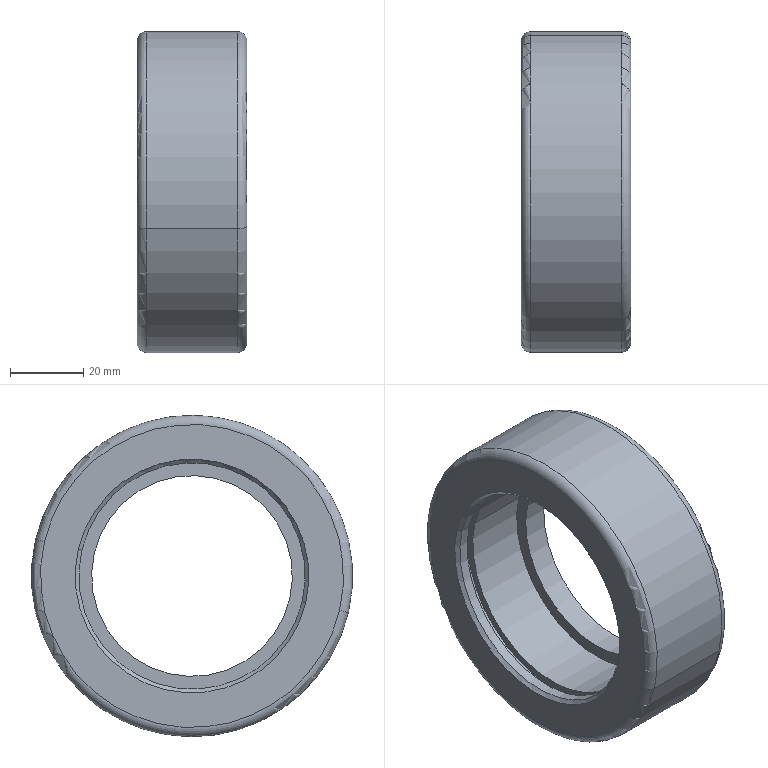Component | SolidWorks | GuideWheelAssembly-1_GuideWheel-2 | 1 solid | 21 faces | box 30 x 88 x 88 mm | volume 94633 mm3 | cylinder 10 | plane 5 | torus 4 | cone 2 | commonest cylinder face diameters 62 x4 66.2 x2 55 x2 88 x2 | material Nylon 101
build123d program:
from build123d import *

# Parameters (mm, degrees)
SKETCH1_R           = 44
BOSS_EXTRUDE1_DEPTH = 30
SKETCH4_R           = 31
CUT_EXTRUDE2_DEPTH  = 67.34
SKETCH5_R           = 27.5
CUT_EXTRUDE3_DEPTH  = 70.08
SKETCH6_R           = 33.1
CUT_EXTRUDE4_DEPTH  = 2.2
CHAMFER1_SIZE       = 1
FILLET1_R           = 2.5


with BuildPart() as part:
    # Sketch1 → Boss-Extrude1 (new body)
    with BuildSketch(Plane.XY):
        Circle(SKETCH1_R)
    extrude(amount=BOSS_EXTRUDE1_DEPTH)

    # Sketch4 → Cut-Extrude2 (cut, through all)
    with BuildSketch(Plane.XY.offset(7)):
        Circle(SKETCH4_R)
    extrude(amount=CUT_EXTRUDE2_DEPTH, mode=Mode.SUBTRACT)

    # Sketch5 → Cut-Extrude3 (cut, through all)
    with BuildSketch(Plane(origin=(0, 0, 0), x_dir=(-1, 0, 0), z_dir=(0, 0, -1))):
        Circle(SKETCH5_R)
    extrude(amount=-CUT_EXTRUDE3_DEPTH, mode=Mode.SUBTRACT)

    # Sketch6 → Cut-Extrude4 (cut)
    with BuildSketch(Plane.XY.offset(24)):
        Circle(SKETCH6_R)
    extrude(amount=CUT_EXTRUDE4_DEPTH, mode=Mode.SUBTRACT)

    # Chamfer1
    chamfer1_edges = [part.edges().sort_by_distance(p)[0] for p in [
        (-31, 0, 30),
    ]]
    chamfer(chamfer1_edges, length=CHAMFER1_SIZE)

    # Fillet1
    fillet1_edges = [part.edges().sort_by_distance(p)[0] for p in [
        (-44, 0, 0),
        (-44, 0, 30),
    ]]
    fillet(fillet1_edges, radius=FILLET1_R)


solid = part.part

# Placed as in the assembly
solid = solid.moved(Location((-540, 0, 25), (0, -90, 0)))
STEP:
#1=COLOUR_RGB('',0.7922,0.8196,0.9333);
#2=FILL_AREA_STYLE_COLOUR('',#1);
#3=FILL_AREA_STYLE('',(#2));
#4=SURFACE_STYLE_FILL_AREA(#3);
#5=SURFACE_SIDE_STYLE('',(#4));
#6=SURFACE_STYLE_USAGE(.BOTH.,#5);
#7=PRESENTATION_STYLE_ASSIGNMENT((#6));
#8=CARTESIAN_POINT('',(-21.26,-1.591,0.6126));
#9=VERTEX_POINT('',#8);
#10=CARTESIAN_POINT('',(-21.26,1.591,1.356));
#11=VERTEX_POINT('',#10);
#12=CARTESIAN_POINT('',(-21.26,-0.,0.9843));
#13=DIRECTION('',(1.,0.,0.));
#14=DIRECTION('',(0.,0.9738,0.2275));
#15=AXIS2_PLACEMENT_3D('',#12,#13,#14);
#16=CIRCLE('',#15,1.634);
#17=EDGE_CURVE('',#9,#11,#16,.T.);
#18=ORIENTED_EDGE('',*,*,#17,.F.);
#19=CARTESIAN_POINT('',(-21.358,-1.687,0.5902));
#20=VERTEX_POINT('',#19);
#21=CARTESIAN_POINT('',(-21.358,-1.591,0.6126));
#22=DIRECTION('',(0.,0.2275,-0.9738));
#23=DIRECTION('',(0.,0.9738,0.2275));
#24=AXIS2_PLACEMENT_3D('',#21,#22,#23);
#25=CIRCLE('',#24,0.09843);
#26=EDGE_CURVE('',#9,#20,#25,.T.);
#27=ORIENTED_EDGE('',*,*,#26,.T.);
#28=CARTESIAN_POINT('',(-21.358,1.687,1.378));
#29=VERTEX_POINT('',#28);
#30=CARTESIAN_POINT('',(-21.358,-0.,0.9843));
#31=DIRECTION('',(-1.,0.,0.));
#32=DIRECTION('',(0.,0.9738,0.2275));
#33=AXIS2_PLACEMENT_3D('',#30,#31,#32);
#34=CIRCLE('',#33,1.732);
#35=EDGE_CURVE('',#29,#20,#34,.T.);
#36=ORIENTED_EDGE('',*,*,#35,.F.);
#37=CARTESIAN_POINT('',(-21.358,1.591,1.356));
#38=DIRECTION('',(0.,-0.2275,0.9738));
#39=DIRECTION('',(0.,-0.9738,-0.2275));
#40=AXIS2_PLACEMENT_3D('',#37,#38,#39);
#41=CIRCLE('',#40,0.09843);
#42=EDGE_CURVE('',#11,#29,#41,.T.);
#43=ORIENTED_EDGE('',*,*,#42,.F.);
#44=EDGE_LOOP('',(#18,#27,#36,#43));
#45=FACE_OUTER_BOUND('',#44,.T.);
#46=CARTESIAN_POINT('',(-21.358,-0.,0.9843));
#47=DIRECTION('',(-1.,0.,0.));
#48=DIRECTION('',(0.,0.9738,0.2275));
#49=AXIS2_PLACEMENT_3D('',#46,#47,#48);
#50=TOROIDAL_SURFACE('',#49,1.634,0.09843);
#51=ADVANCED_FACE('',(#45),#50,.T.);
#52=CARTESIAN_POINT('',(-22.343,-1.687,0.5902));
#53=VERTEX_POINT('',#52);
#54=CARTESIAN_POINT('',(-22.343,1.687,1.378));
#55=VERTEX_POINT('',#54);
#56=CARTESIAN_POINT('',(-22.343,-0.,0.9843));
#57=DIRECTION('',(1.,0.,0.));
#58=DIRECTION('',(0.,0.9738,0.2275));
#59=AXIS2_PLACEMENT_3D('',#56,#57,#58);
#60=CIRCLE('',#59,1.732);
#61=EDGE_CURVE('',#53,#55,#60,.T.);
#62=ORIENTED_EDGE('',*,*,#61,.F.);
#63=CARTESIAN_POINT('',(-22.441,-1.591,0.6126));
#64=VERTEX_POINT('',#63);
#65=CARTESIAN_POINT('',(-22.343,-1.591,0.6126));
#66=DIRECTION('',(0.,0.2275,-0.9738));
#67=DIRECTION('',(0.,0.9738,0.2275));
#68=AXIS2_PLACEMENT_3D('',#65,#66,#67);
#69=CIRCLE('',#68,0.09843);
#70=EDGE_CURVE('',#53,#64,#69,.T.);
#71=ORIENTED_EDGE('',*,*,#70,.T.);
#72=CARTESIAN_POINT('',(-22.441,1.591,1.356));
#73=VERTEX_POINT('',#72);
#74=CARTESIAN_POINT('',(-22.441,-0.,0.9843));
#75=DIRECTION('',(-1.,0.,0.));
#76=DIRECTION('',(0.,0.9738,0.2275));
#77=AXIS2_PLACEMENT_3D('',#74,#75,#76);
#78=CIRCLE('',#77,1.634);
#79=EDGE_CURVE('',#73,#64,#78,.T.);
#80=ORIENTED_EDGE('',*,*,#79,.F.);
#81=CARTESIAN_POINT('',(-22.343,1.591,1.356));
#82=DIRECTION('',(0.,-0.2275,0.9738));
#83=DIRECTION('',(0.,-0.9738,-0.2275));
#84=AXIS2_PLACEMENT_3D('',#81,#82,#83);
#85=CIRCLE('',#84,0.09843);
#86=EDGE_CURVE('',#55,#73,#85,.T.);
#87=ORIENTED_EDGE('',*,*,#86,.F.);
#88=EDGE_LOOP('',(#62,#71,#80,#87));
#89=FACE_OUTER_BOUND('',#88,.T.);
#90=CARTESIAN_POINT('',(-22.343,-0.,0.9843));
#91=DIRECTION('',(-1.,0.,0.));
#92=DIRECTION('',(0.,0.9738,0.2275));
#93=AXIS2_PLACEMENT_3D('',#90,#91,#92);
#94=TOROIDAL_SURFACE('',#93,1.634,0.09843);
#95=ADVANCED_FACE('',(#89),#94,.T.);
#96=CARTESIAN_POINT('',(-22.402,-1.188,0.7066));
#97=VERTEX_POINT('',#96);
#98=CARTESIAN_POINT('',(-22.402,1.188,1.262));
#99=VERTEX_POINT('',#98);
#100=CARTESIAN_POINT('',(-22.402,-0.,0.9843));
#101=DIRECTION('',(-1.,0.,0.));
#102=DIRECTION('',(0.,0.9738,0.2275));
#103=AXIS2_PLACEMENT_3D('',#100,#101,#102);
#104=CIRCLE('',#103,1.22);
#105=EDGE_CURVE('',#97,#99,#104,.T.);
#106=ORIENTED_EDGE('',*,*,#105,.F.);
#107=CARTESIAN_POINT('',(-22.441,-1.227,0.6977));
#108=VERTEX_POINT('',#107);
#109=CARTESIAN_POINT('',(-22.402,-1.188,0.7066));
#110=DIRECTION('',(-0.7071,-0.6886,-0.1608));
#111=VECTOR('',#110,39.37);
#112=LINE('',#109,#111);
#113=EDGE_CURVE('',#97,#108,#112,.T.);
#114=ORIENTED_EDGE('',*,*,#113,.T.);
#115=CARTESIAN_POINT('',(-22.441,1.227,1.271));
#116=VERTEX_POINT('',#115);
#117=CARTESIAN_POINT('',(-22.441,-0.,0.9843));
#118=DIRECTION('',(1.,0.,0.));
#119=DIRECTION('',(0.,0.9738,0.2275));
#120=AXIS2_PLACEMENT_3D('',#117,#118,#119);
#121=CIRCLE('',#120,1.26);
#122=EDGE_CURVE('',#116,#108,#121,.T.);
#123=ORIENTED_EDGE('',*,*,#122,.F.);
#124=CARTESIAN_POINT('',(-22.402,1.188,1.262));
#125=DIRECTION('',(-0.7071,0.6886,0.1608));
#126=VECTOR('',#125,39.37);
#127=LINE('',#124,#126);
#128=EDGE_CURVE('',#99,#116,#127,.T.);
#129=ORIENTED_EDGE('',*,*,#128,.F.);
#130=EDGE_LOOP('',(#106,#114,#123,#129));
#131=FACE_OUTER_BOUND('',#130,.T.);
#132=CARTESIAN_POINT('',(-22.402,-0.,0.9843));
#133=DIRECTION('',(-1.,0.,0.));
#134=DIRECTION('',(0.,0.9738,0.2275));
#135=AXIS2_PLACEMENT_3D('',#132,#133,#134);
#136=CONICAL_SURFACE('',#135,1.22,0.7854);
#137=ADVANCED_FACE('',(#131),#136,.F.);
#138=CARTESIAN_POINT('',(-22.291,-1.269,0.6878));
#139=VERTEX_POINT('',#138);
#140=CARTESIAN_POINT('',(-22.291,1.269,1.281));
#141=VERTEX_POINT('',#140);
#142=CARTESIAN_POINT('',(-22.291,-0.,0.9843));
#143=DIRECTION('',(-1.,0.,0.));
#144=DIRECTION('',(0.,0.9738,0.2275));
#145=AXIS2_PLACEMENT_3D('',#142,#143,#144);
#146=CIRCLE('',#145,1.303);
#147=EDGE_CURVE('',#139,#141,#146,.T.);
#148=ORIENTED_EDGE('',*,*,#147,.T.);
#149=CARTESIAN_POINT('',(-22.205,1.269,1.281));
#150=VERTEX_POINT('',#149);
#151=CARTESIAN_POINT('',(-22.291,1.269,1.281));
#152=DIRECTION('',(1.,0.,0.));
#153=VECTOR('',#152,39.37);
#154=LINE('',#151,#153);
#155=EDGE_CURVE('',#141,#150,#154,.T.);
#156=ORIENTED_EDGE('',*,*,#155,.T.);
#157=CARTESIAN_POINT('',(-22.205,-1.269,0.6878));
#158=VERTEX_POINT('',#157);
#159=CARTESIAN_POINT('',(-22.205,-0.,0.9843));
#160=DIRECTION('',(-1.,0.,0.));
#161=DIRECTION('',(0.,0.9738,0.2275));
#162=AXIS2_PLACEMENT_3D('',#159,#160,#161);
#163=CIRCLE('',#162,1.303);
#164=EDGE_CURVE('',#158,#150,#163,.T.);
#165=ORIENTED_EDGE('',*,*,#164,.F.);
#166=CARTESIAN_POINT('',(-22.291,-1.269,0.6878));
#167=DIRECTION('',(1.,0.,0.));
#168=VECTOR('',#167,39.37);
#169=LINE('',#166,#168);
#170=EDGE_CURVE('',#139,#158,#169,.T.);
#171=ORIENTED_EDGE('',*,*,#170,.F.);
#172=EDGE_LOOP('',(#148,#156,#165,#171));
#173=FACE_OUTER_BOUND('',#172,.T.);
#174=CARTESIAN_POINT('',(-22.291,-0.,0.9843));
#175=DIRECTION('',(1.,0.,0.));
#176=DIRECTION('',(0.,-0.9738,-0.2275));
#177=AXIS2_PLACEMENT_3D('',#174,#175,#176);
#178=CYLINDRICAL_SURFACE('',#177,1.303);
#179=ADVANCED_FACE('',(#173),#178,.F.);
#180=CARTESIAN_POINT('',(-21.535,-1.054,0.738));
#181=VERTEX_POINT('',#180);
#182=CARTESIAN_POINT('',(-21.535,1.054,1.231));
#183=VERTEX_POINT('',#182);
#184=CARTESIAN_POINT('',(-21.535,-0.,0.9843));
#185=DIRECTION('',(-1.,0.,0.));
#186=DIRECTION('',(0.,0.9738,0.2275));
#187=AXIS2_PLACEMENT_3D('',#184,#185,#186);
#188=CIRCLE('',#187,1.083);
#189=EDGE_CURVE('',#181,#183,#188,.T.);
#190=ORIENTED_EDGE('',*,*,#189,.T.);
#191=CARTESIAN_POINT('',(-21.26,1.054,1.231));
#192=VERTEX_POINT('',#191);
#193=CARTESIAN_POINT('',(-22.441,1.054,1.231));
#194=DIRECTION('',(1.,0.,0.));
#195=VECTOR('',#194,39.37);
#196=LINE('',#193,#195);
#197=EDGE_CURVE('',#183,#192,#196,.T.);
#198=ORIENTED_EDGE('',*,*,#197,.T.);
#199=CARTESIAN_POINT('',(-21.26,-1.054,0.738));
#200=VERTEX_POINT('',#199);
#201=CARTESIAN_POINT('',(-21.26,-0.,0.9843));
#202=DIRECTION('',(1.,0.,0.));
#203=DIRECTION('',(0.,-0.9738,-0.2275));
#204=AXIS2_PLACEMENT_3D('',#201,#202,#203);
#205=CIRCLE('',#204,1.083);
#206=EDGE_CURVE('',#192,#200,#205,.T.);
#207=ORIENTED_EDGE('',*,*,#206,.T.);
#208=CARTESIAN_POINT('',(-22.441,-1.054,0.738));
#209=DIRECTION('',(1.,0.,0.));
#210=VECTOR('',#209,39.37);
#211=LINE('',#208,#210);
#212=EDGE_CURVE('',#181,#200,#211,.T.);
#213=ORIENTED_EDGE('',*,*,#212,.F.);
#214=EDGE_LOOP('',(#190,#198,#207,#213));
#215=FACE_OUTER_BOUND('',#214,.T.);
#216=CARTESIAN_POINT('',(-22.441,-0.,0.9843));
#217=DIRECTION('',(1.,0.,0.));
#218=DIRECTION('',(0.,-0.9738,-0.2275));
#219=AXIS2_PLACEMENT_3D('',#216,#217,#218);
#220=CYLINDRICAL_SURFACE('',#219,1.083);
#221=ADVANCED_FACE('',(#215),#220,.F.);
#222=ORIENTED_EDGE('',*,*,#105,.T.);
#223=CARTESIAN_POINT('',(-22.291,1.188,1.262));
#224=VERTEX_POINT('',#223);
#225=CARTESIAN_POINT('',(-22.441,1.188,1.262));
#226=DIRECTION('',(1.,0.,0.));
#227=VECTOR('',#226,39.37);
#228=LINE('',#225,#227);
#229=EDGE_CURVE('',#99,#224,#228,.T.);
#230=ORIENTED_EDGE('',*,*,#229,.T.);
#231=CARTESIAN_POINT('',(-22.291,-1.188,0.7066));
#232=VERTEX_POINT('',#231);
#233=CARTESIAN_POINT('',(-22.291,-0.,0.9843));
#234=DIRECTION('',(-1.,0.,0.));
#235=DIRECTION('',(0.,0.9738,0.2275));
#236=AXIS2_PLACEMENT_3D('',#233,#234,#235);
#237=CIRCLE('',#236,1.22);
#238=EDGE_CURVE('',#232,#224,#237,.T.);
#239=ORIENTED_EDGE('',*,*,#238,.F.);
#240=CARTESIAN_POINT('',(-22.441,-1.188,0.7066));
#241=DIRECTION('',(1.,0.,0.));
#242=VECTOR('',#241,39.37);
#243=LINE('',#240,#242);
#244=EDGE_CURVE('',#97,#232,#243,.T.);
#245=ORIENTED_EDGE('',*,*,#244,.F.);
#246=EDGE_LOOP('',(#222,#230,#239,#245));
#247=FACE_OUTER_BOUND('',#246,.T.);
#248=CARTESIAN_POINT('',(-22.441,-0.,0.9843));
#249=DIRECTION('',(1.,0.,0.));
#250=DIRECTION('',(0.,-0.9738,-0.2275));
#251=AXIS2_PLACEMENT_3D('',#248,#249,#250);
#252=CYLINDRICAL_SURFACE('',#251,1.22);
#253=ADVANCED_FACE('',(#247),#252,.F.);
#254=ORIENTED_EDGE('',*,*,#61,.T.);
#255=CARTESIAN_POINT('',(-22.441,1.687,1.378));
#256=DIRECTION('',(1.,0.,0.));
#257=VECTOR('',#256,39.37);
#258=LINE('',#255,#257);
#259=EDGE_CURVE('',#55,#29,#258,.T.);
#260=ORIENTED_EDGE('',*,*,#259,.T.);
#261=ORIENTED_EDGE('',*,*,#35,.T.);
#262=CARTESIAN_POINT('',(-22.441,-1.687,0.5902));
#263=DIRECTION('',(1.,0.,0.));
#264=VECTOR('',#263,39.37);
#265=LINE('',#262,#264);
#266=EDGE_CURVE('',#53,#20,#265,.T.);
#267=ORIENTED_EDGE('',*,*,#266,.F.);
#268=EDGE_LOOP('',(#254,#260,#261,#267));
#269=FACE_OUTER_BOUND('',#268,.T.);
#270=CARTESIAN_POINT('',(-22.441,-0.,0.9843));
#271=DIRECTION('',(1.,0.,0.));
#272=DIRECTION('',(0.,-0.9738,-0.2275));
#273=AXIS2_PLACEMENT_3D('',#270,#271,#272);
#274=CYLINDRICAL_SURFACE('',#273,1.732);
#275=ADVANCED_FACE('',(#269),#274,.T.);
#276=CARTESIAN_POINT('',(-22.205,-1.188,0.7066));
#277=VERTEX_POINT('',#276);
#278=CARTESIAN_POINT('',(-22.205,1.188,1.262));
#279=VERTEX_POINT('',#278);
#280=CARTESIAN_POINT('',(-22.205,-0.,0.9843));
#281=DIRECTION('',(-1.,0.,0.));
#282=DIRECTION('',(0.,0.9738,0.2275));
#283=AXIS2_PLACEMENT_3D('',#280,#281,#282);
#284=CIRCLE('',#283,1.22);
#285=EDGE_CURVE('',#277,#279,#284,.T.);
#286=ORIENTED_EDGE('',*,*,#285,.T.);
#287=CARTESIAN_POINT('',(-21.535,1.188,1.262));
#288=VERTEX_POINT('',#287);
#289=CARTESIAN_POINT('',(-22.441,1.188,1.262));
#290=DIRECTION('',(1.,0.,0.));
#291=VECTOR('',#290,39.37);
#292=LINE('',#289,#291);
#293=EDGE_CURVE('',#279,#288,#292,.T.);
#294=ORIENTED_EDGE('',*,*,#293,.T.);
#295=CARTESIAN_POINT('',(-21.535,-1.188,0.7066));
#296=VERTEX_POINT('',#295);
#297=CARTESIAN_POINT('',(-21.535,-0.,0.9843));
#298=DIRECTION('',(-1.,0.,0.));
#299=DIRECTION('',(0.,0.9738,0.2275));
#300=AXIS2_PLACEMENT_3D('',#297,#298,#299);
#301=CIRCLE('',#300,1.22);
#302=EDGE_CURVE('',#296,#288,#301,.T.);
#303=ORIENTED_EDGE('',*,*,#302,.F.);
#304=CARTESIAN_POINT('',(-22.441,-1.188,0.7066));
#305=DIRECTION('',(1.,0.,0.));
#306=VECTOR('',#305,39.37);
#307=LINE('',#304,#306);
#308=EDGE_CURVE('',#277,#296,#307,.T.);
#309=ORIENTED_EDGE('',*,*,#308,.F.);
#310=EDGE_LOOP('',(#286,#294,#303,#309));
#311=FACE_OUTER_BOUND('',#310,.T.);
#312=CARTESIAN_POINT('',(-22.441,-0.,0.9843));
#313=DIRECTION('',(1.,0.,0.));
#314=DIRECTION('',(0.,-0.9738,-0.2275));
#315=AXIS2_PLACEMENT_3D('',#312,#313,#314);
#316=CYLINDRICAL_SURFACE('',#315,1.22);
#317=ADVANCED_FACE('',(#311),#316,.F.);
#318=ORIENTED_EDGE('',*,*,#293,.F.);
#319=CARTESIAN_POINT('',(-22.205,-0.,0.9843));
#320=DIRECTION('',(-1.,0.,0.));
#321=DIRECTION('',(0.,0.9738,0.2275));
#322=AXIS2_PLACEMENT_3D('',#319,#320,#321);
#323=CIRCLE('',#322,1.22);
#324=EDGE_CURVE('',#279,#277,#323,.T.);
#325=ORIENTED_EDGE('',*,*,#324,.T.);
#326=ORIENTED_EDGE('',*,*,#308,.T.);
#327=CARTESIAN_POINT('',(-21.535,-0.,0.9843));
#328=DIRECTION('',(-1.,0.,0.));
#329=DIRECTION('',(0.,0.9738,0.2275));
#330=AXIS2_PLACEMENT_3D('',#327,#328,#329);
#331=CIRCLE('',#330,1.22);
#332=EDGE_CURVE('',#288,#296,#331,.T.);
#333=ORIENTED_EDGE('',*,*,#332,.F.);
#334=EDGE_LOOP('',(#318,#325,#326,#333));
#335=FACE_OUTER_BOUND('',#334,.T.);
#336=CARTESIAN_POINT('',(-22.441,-0.,0.9843));
#337=DIRECTION('',(1.,0.,0.));
#338=DIRECTION('',(0.,-0.9738,-0.2275));
#339=AXIS2_PLACEMENT_3D('',#336,#337,#338);
#340=CYLINDRICAL_SURFACE('',#339,1.22);
#341=ADVANCED_FACE('',(#335),#340,.F.);
#342=ORIENTED_EDGE('',*,*,#79,.T.);
#343=CARTESIAN_POINT('',(-22.441,-0.,0.9843));
#344=DIRECTION('',(-1.,0.,0.));
#345=DIRECTION('',(0.,0.9738,0.2275));
#346=AXIS2_PLACEMENT_3D('',#343,#344,#345);
#347=CIRCLE('',#346,1.634);
#348=EDGE_CURVE('',#64,#73,#347,.T.);
#349=ORIENTED_EDGE('',*,*,#348,.T.);
#350=EDGE_LOOP('',(#342,#349));
#351=FACE_OUTER_BOUND('',#350,.T.);
#352=ORIENTED_EDGE('',*,*,#122,.T.);
#353=CARTESIAN_POINT('',(-22.441,-0.,0.9843));
#354=DIRECTION('',(1.,0.,0.));
#355=DIRECTION('',(0.,0.9738,0.2275));
#356=AXIS2_PLACEMENT_3D('',#353,#354,#355);
#357=CIRCLE('',#356,1.26);
#358=EDGE_CURVE('',#108,#116,#357,.T.);
#359=ORIENTED_EDGE('',*,*,#358,.T.);
#360=EDGE_LOOP('',(#352,#359));
#361=FACE_BOUND('',#360,.T.);
#362=CARTESIAN_POINT('',(-22.441,-0.,0.9843));
#363=DIRECTION('',(-1.,0.,0.));
#364=DIRECTION('',(0.,0.9738,0.2275));
#365=AXIS2_PLACEMENT_3D('',#362,#363,#364);
#366=PLANE('',#365);
#367=ADVANCED_FACE('',(#351,#361),#366,.T.);
#368=ORIENTED_EDGE('',*,*,#259,.F.);
#369=CARTESIAN_POINT('',(-22.343,-0.,0.9843));
#370=DIRECTION('',(1.,0.,0.));
#371=DIRECTION('',(0.,0.9738,0.2275));
#372=AXIS2_PLACEMENT_3D('',#369,#370,#371);
#373=CIRCLE('',#372,1.732);
#374=EDGE_CURVE('',#55,#53,#373,.T.);
#375=ORIENTED_EDGE('',*,*,#374,.T.);
#376=ORIENTED_EDGE('',*,*,#266,.T.);
#377=CARTESIAN_POINT('',(-21.358,-0.,0.9843));
#378=DIRECTION('',(-1.,0.,0.));
#379=DIRECTION('',(0.,0.9738,0.2275));
#380=AXIS2_PLACEMENT_3D('',#377,#378,#379);
#381=CIRCLE('',#380,1.732);
#382=EDGE_CURVE('',#20,#29,#381,.T.);
#383=ORIENTED_EDGE('',*,*,#382,.T.);
#384=EDGE_LOOP('',(#368,#375,#376,#383));
#385=FACE_OUTER_BOUND('',#384,.T.);
#386=CARTESIAN_POINT('',(-22.441,-0.,0.9843));
#387=DIRECTION('',(1.,0.,0.));
#388=DIRECTION('',(0.,-0.9738,-0.2275));
#389=AXIS2_PLACEMENT_3D('',#386,#387,#388);
#390=CYLINDRICAL_SURFACE('',#389,1.732);
#391=ADVANCED_FACE('',(#385),#390,.T.);
#392=CARTESIAN_POINT('',(-21.26,-0.,0.9843));
#393=DIRECTION('',(1.,0.,0.));
#394=DIRECTION('',(0.,0.9738,0.2275));
#395=AXIS2_PLACEMENT_3D('',#392,#393,#394);
#396=CIRCLE('',#395,1.634);
#397=EDGE_CURVE('',#11,#9,#396,.T.);
#398=ORIENTED_EDGE('',*,*,#397,.T.);
#399=ORIENTED_EDGE('',*,*,#17,.T.);
#400=EDGE_LOOP('',(#398,#399));
#401=FACE_OUTER_BOUND('',#400,.T.);
#402=CARTESIAN_POINT('',(-21.26,-0.,0.9843));
#403=DIRECTION('',(1.,0.,0.));
#404=DIRECTION('',(0.,-0.9738,-0.2275));
#405=AXIS2_PLACEMENT_3D('',#402,#403,#404);
#406=CIRCLE('',#405,1.083);
#407=EDGE_CURVE('',#200,#192,#406,.T.);
#408=ORIENTED_EDGE('',*,*,#407,.F.);
#409=ORIENTED_EDGE('',*,*,#206,.F.);
#410=EDGE_LOOP('',(#408,#409));
#411=FACE_BOUND('',#410,.T.);
#412=CARTESIAN_POINT('',(-21.26,-0.,0.9843));
#413=DIRECTION('',(-1.,0.,0.));
#414=DIRECTION('',(0.,0.9738,0.2275));
#415=AXIS2_PLACEMENT_3D('',#412,#413,#414);
#416=PLANE('',#415);
#417=ADVANCED_FACE('',(#401,#411),#416,.F.);
#418=ORIENTED_EDGE('',*,*,#229,.F.);
#419=CARTESIAN_POINT('',(-22.402,-0.,0.9843));
#420=DIRECTION('',(-1.,0.,0.));
#421=DIRECTION('',(0.,0.9738,0.2275));
#422=AXIS2_PLACEMENT_3D('',#419,#420,#421);
#423=CIRCLE('',#422,1.22);
#424=EDGE_CURVE('',#99,#97,#423,.T.);
#425=ORIENTED_EDGE('',*,*,#424,.T.);
#426=ORIENTED_EDGE('',*,*,#244,.T.);
#427=CARTESIAN_POINT('',(-22.291,-0.,0.9843));
#428=DIRECTION('',(-1.,0.,0.));
#429=DIRECTION('',(0.,0.9738,0.2275));
#430=AXIS2_PLACEMENT_3D('',#427,#428,#429);
#431=CIRCLE('',#430,1.22);
#432=EDGE_CURVE('',#224,#232,#431,.T.);
#433=ORIENTED_EDGE('',*,*,#432,.F.);
#434=EDGE_LOOP('',(#418,#425,#426,#433));
#435=FACE_OUTER_BOUND('',#434,.T.);
#436=CARTESIAN_POINT('',(-22.441,-0.,0.9843));
#437=DIRECTION('',(1.,0.,0.));
#438=DIRECTION('',(0.,-0.9738,-0.2275));
#439=AXIS2_PLACEMENT_3D('',#436,#437,#438);
#440=CYLINDRICAL_SURFACE('',#439,1.22);
#441=ADVANCED_FACE('',(#435),#440,.F.);
#442=ORIENTED_EDGE('',*,*,#189,.F.);
#443=CARTESIAN_POINT('',(-21.535,-0.,0.9843));
#444=DIRECTION('',(-1.,0.,0.));
#445=DIRECTION('',(0.,0.9738,0.2275));
#446=AXIS2_PLACEMENT_3D('',#443,#444,#445);
#447=CIRCLE('',#446,1.083);
#448=EDGE_CURVE('',#183,#181,#447,.T.);
#449=ORIENTED_EDGE('',*,*,#448,.F.);
#450=EDGE_LOOP('',(#442,#449));
#451=FACE_BOUND('',#450,.T.);
#452=ORIENTED_EDGE('',*,*,#302,.T.);
#453=ORIENTED_EDGE('',*,*,#332,.T.);
#454=EDGE_LOOP('',(#452,#453));
#455=FACE_OUTER_BOUND('',#454,.T.);
#456=CARTESIAN_POINT('',(-21.535,-0.,0.9843));
#457=DIRECTION('',(-1.,0.,0.));
#458=DIRECTION('',(0.,0.9738,0.2275));
#459=AXIS2_PLACEMENT_3D('',#456,#457,#458);
#460=PLANE('',#459);
#461=ADVANCED_FACE('',(#451,#455),#460,.T.);
#462=ORIENTED_EDGE('',*,*,#197,.F.);
#463=ORIENTED_EDGE('',*,*,#448,.T.);
#464=ORIENTED_EDGE('',*,*,#212,.T.);
#465=ORIENTED_EDGE('',*,*,#407,.T.);
#466=EDGE_LOOP('',(#462,#463,#464,#465));
#467=FACE_OUTER_BOUND('',#466,.T.);
#468=CARTESIAN_POINT('',(-22.441,-0.,0.9843));
#469=DIRECTION('',(1.,0.,0.));
#470=DIRECTION('',(0.,-0.9738,-0.2275));
#471=AXIS2_PLACEMENT_3D('',#468,#469,#470);
#472=CYLINDRICAL_SURFACE('',#471,1.083);
#473=ADVANCED_FACE('',(#467),#472,.F.);
#474=ORIENTED_EDGE('',*,*,#155,.F.);
#475=CARTESIAN_POINT('',(-22.291,-0.,0.9843));
#476=DIRECTION('',(-1.,0.,0.));
#477=DIRECTION('',(0.,0.9738,0.2275));
#478=AXIS2_PLACEMENT_3D('',#475,#476,#477);
#479=CIRCLE('',#478,1.303);
#480=EDGE_CURVE('',#141,#139,#479,.T.);
#481=ORIENTED_EDGE('',*,*,#480,.T.);
#482=ORIENTED_EDGE('',*,*,#170,.T.);
#483=CARTESIAN_POINT('',(-22.205,-0.,0.9843));
#484=DIRECTION('',(-1.,0.,0.));
#485=DIRECTION('',(0.,0.9738,0.2275));
#486=AXIS2_PLACEMENT_3D('',#483,#484,#485);
#487=CIRCLE('',#486,1.303);
#488=EDGE_CURVE('',#150,#158,#487,.T.);
#489=ORIENTED_EDGE('',*,*,#488,.F.);
#490=EDGE_LOOP('',(#474,#481,#482,#489));
#491=FACE_OUTER_BOUND('',#490,.T.);
#492=CARTESIAN_POINT('',(-22.291,-0.,0.9843));
#493=DIRECTION('',(1.,0.,0.));
#494=DIRECTION('',(0.,-0.9738,-0.2275));
#495=AXIS2_PLACEMENT_3D('',#492,#493,#494);
#496=CYLINDRICAL_SURFACE('',#495,1.303);
#497=ADVANCED_FACE('',(#491),#496,.F.);
#498=ORIENTED_EDGE('',*,*,#238,.T.);
#499=ORIENTED_EDGE('',*,*,#432,.T.);
#500=EDGE_LOOP('',(#498,#499));
#501=FACE_BOUND('',#500,.T.);
#502=ORIENTED_EDGE('',*,*,#147,.F.);
#503=ORIENTED_EDGE('',*,*,#480,.F.);
#504=EDGE_LOOP('',(#502,#503));
#505=FACE_OUTER_BOUND('',#504,.T.);
#506=CARTESIAN_POINT('',(-22.291,-0.,0.9843));
#507=DIRECTION('',(-1.,0.,0.));
#508=DIRECTION('',(0.,0.9738,0.2275));
#509=AXIS2_PLACEMENT_3D('',#506,#507,#508);
#510=PLANE('',#509);
#511=ADVANCED_FACE('',(#501,#505),#510,.F.);
#512=ORIENTED_EDGE('',*,*,#285,.F.);
#513=ORIENTED_EDGE('',*,*,#324,.F.);
#514=EDGE_LOOP('',(#512,#513));
#515=FACE_BOUND('',#514,.T.);
#516=ORIENTED_EDGE('',*,*,#164,.T.);
#517=ORIENTED_EDGE('',*,*,#488,.T.);
#518=EDGE_LOOP('',(#516,#517));
#519=FACE_OUTER_BOUND('',#518,.T.);
#520=CARTESIAN_POINT('',(-22.205,-0.,0.9843));
#521=DIRECTION('',(-1.,0.,0.));
#522=DIRECTION('',(0.,0.9738,0.2275));
#523=AXIS2_PLACEMENT_3D('',#520,#521,#522);
#524=PLANE('',#523);
#525=ADVANCED_FACE('',(#515,#519),#524,.T.);
#526=ORIENTED_EDGE('',*,*,#113,.F.);
#527=ORIENTED_EDGE('',*,*,#424,.F.);
#528=ORIENTED_EDGE('',*,*,#128,.T.);
#529=ORIENTED_EDGE('',*,*,#358,.F.);
#530=EDGE_LOOP('',(#526,#527,#528,#529));
#531=FACE_OUTER_BOUND('',#530,.T.);
#532=CARTESIAN_POINT('',(-22.402,-0.,0.9843));
#533=DIRECTION('',(-1.,0.,0.));
#534=DIRECTION('',(0.,0.9738,0.2275));
#535=AXIS2_PLACEMENT_3D('',#532,#533,#534);
#536=CONICAL_SURFACE('',#535,1.22,0.7854);
#537=ADVANCED_FACE('',(#531),#536,.F.);
#538=ORIENTED_EDGE('',*,*,#70,.F.);
#539=ORIENTED_EDGE('',*,*,#374,.F.);
#540=ORIENTED_EDGE('',*,*,#86,.T.);
#541=ORIENTED_EDGE('',*,*,#348,.F.);
#542=EDGE_LOOP('',(#538,#539,#540,#541));
#543=FACE_OUTER_BOUND('',#542,.T.);
#544=CARTESIAN_POINT('',(-22.343,-0.,0.9843));
#545=DIRECTION('',(-1.,0.,0.));
#546=DIRECTION('',(0.,0.9738,0.2275));
#547=AXIS2_PLACEMENT_3D('',#544,#545,#546);
#548=TOROIDAL_SURFACE('',#547,1.634,0.09843);
#549=ADVANCED_FACE('',(#543),#548,.T.);
#550=ORIENTED_EDGE('',*,*,#26,.F.);
#551=ORIENTED_EDGE('',*,*,#397,.F.);
#552=ORIENTED_EDGE('',*,*,#42,.T.);
#553=ORIENTED_EDGE('',*,*,#382,.F.);
#554=EDGE_LOOP('',(#550,#551,#552,#553));
#555=FACE_OUTER_BOUND('',#554,.T.);
#556=CARTESIAN_POINT('',(-21.358,-0.,0.9843));
#557=DIRECTION('',(-1.,0.,0.));
#558=DIRECTION('',(0.,0.9738,0.2275));
#559=AXIS2_PLACEMENT_3D('',#556,#557,#558);
#560=TOROIDAL_SURFACE('',#559,1.634,0.09843);
#561=ADVANCED_FACE('',(#555),#560,.T.);
#562=CLOSED_SHELL('',(#51,#95,#137,#179,#221,#253,#275,#317,#341,#367,#391,#417,#441,#461,#473,#497,#511,#525,#537,#549,#561));
#563=MANIFOLD_SOLID_BREP('',#562);
#564=STYLED_ITEM('',(#7),#563);
#565=PRESENTATION_LAYER_ASSIGNMENT('','',(#564));
#566=CARTESIAN_POINT('',(0.,0.,0.));
#567=DIRECTION('',(0.,0.,1.));
#568=DIRECTION('',(1.,0.,0.));
#569=AXIS2_PLACEMENT_3D('',#566,#567,#568);
#570=(LENGTH_UNIT()NAMED_UNIT(*)SI_UNIT($,.METRE.));
#571=LENGTH_MEASURE_WITH_UNIT(LENGTH_MEASURE(0.0254),#570);
#572=DIMENSIONAL_EXPONENTS(1.,0.,0.,0.,0.,0.,0.);
#573=(CONVERSION_BASED_UNIT('',#571)LENGTH_UNIT()NAMED_UNIT(#572));
#574=UNCERTAINTY_MEASURE_WITH_UNIT(LENGTH_MEASURE(0.00001),#573,'','');
#575=(NAMED_UNIT(*)PLANE_ANGLE_UNIT()SI_UNIT($,.RADIAN.));
#576=(NAMED_UNIT(*)SI_UNIT($,.STERADIAN.)SOLID_ANGLE_UNIT());
#577=(GEOMETRIC_REPRESENTATION_CONTEXT(3)GLOBAL_UNCERTAINTY_ASSIGNED_CONTEXT((#574))GLOBAL_UNIT_ASSIGNED_CONTEXT((#573,#575,#576))REPRESENTATION_CONTEXT('',''));
#578=ADVANCED_BREP_SHAPE_REPRESENTATION('',(#563,#569),#577);
#579=(LENGTH_UNIT()NAMED_UNIT(*)SI_UNIT($,.METRE.));
#580=LENGTH_MEASURE_WITH_UNIT(LENGTH_MEASURE(0.0254),#579);
#581=DIMENSIONAL_EXPONENTS(1.,0.,0.,0.,0.,0.,0.);
#582=(CONVERSION_BASED_UNIT('',#580)LENGTH_UNIT()NAMED_UNIT(#581));
#583=UNCERTAINTY_MEASURE_WITH_UNIT(LENGTH_MEASURE(0.00001),#582,'','');
#584=(NAMED_UNIT(*)PLANE_ANGLE_UNIT()SI_UNIT($,.RADIAN.));
#585=(NAMED_UNIT(*)SI_UNIT($,.STERADIAN.)SOLID_ANGLE_UNIT());
#586=(GEOMETRIC_REPRESENTATION_CONTEXT(3)GLOBAL_UNCERTAINTY_ASSIGNED_CONTEXT((#583))GLOBAL_UNIT_ASSIGNED_CONTEXT((#582,#584,#585))REPRESENTATION_CONTEXT('',''));
#587=MECHANICAL_DESIGN_GEOMETRIC_PRESENTATION_REPRESENTATION('',(#564),#586);